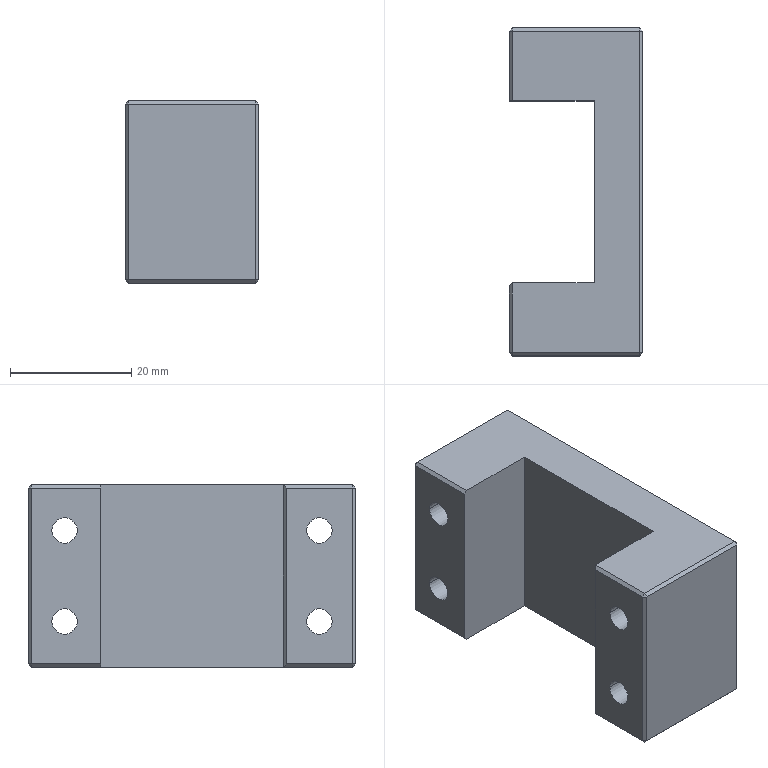Component | SolidWorks | XM-WST05-2009-3 | 1 solid | 41 faces | box 22 x 54 x 30 mm | volume 21772 mm3 | plane 33 | cylinder 8 | commonest cylinder face diameters 4.2 x8
build123d program:
from build123d import *

# Parameters (mm, degrees)
SKETCH1_W           = 54
SKETCH1_H           = 30
BOSS_EXTRUDE1_DEPTH = 22
SKETCH2_W           = 30
SKETCH2_H           = 28
CUT_EXTRUDE1_DEPTH  = 46.967
M5_TAPPED_HOLE1_D   = 4.2
CHAMFER1_SIZE       = 0.5


with BuildPart() as part:
    # Sketch1 → Boss-Extrude1 (new body)
    with BuildSketch(Plane.XY):
        Rectangle(SKETCH1_W, SKETCH1_H)
    extrude(amount=BOSS_EXTRUDE1_DEPTH)

    # Sketch2 → Cut-Extrude1 (cut, through all)
    with BuildSketch(Plane(origin=(0, 15, 0), x_dir=(1, 0, 0), z_dir=(0, 1, 0))):
        with Locations((0, -22)):
            Rectangle(SKETCH2_W, SKETCH2_H)
    extrude(amount=-CUT_EXTRUDE1_DEPTH, mode=Mode.SUBTRACT)

    # M5 Tapped Hole1 (through all)
    with Locations(Plane.XY.offset(22)):
        with Locations((-21, -7.5), (-21, 7.5), (21, 7.5), (21, -7.5)):
            Hole(M5_TAPPED_HOLE1_D / 2)

    # Chamfer1
    chamfer1_edges = [part.edges().sort_by_distance(p)[0] for p in [
        (27, 0, 22),
        (21, 15, 22),
        (21, -15, 22),
        (-21, 15, 22),
        (15, 0, 22),
        (-27, 0, 22),
        (0, 15, 0),
        (27, 0, 0),
        (0, -15, 0),
        (-27, 0, 0),
        (-21, -15, 22),
        (-27, 15, 11),
        (27, 15, 11),
        (27, -15, 11),
        (-27, -15, 11),
    ]]
    chamfer(chamfer1_edges, length=CHAMFER1_SIZE)


solid = part.part

# Placed as in the assembly
solid = solid.moved(Location((-131.071, 48.669, 455.899), (90, -90, 0)))
STEP:
#1=COLOUR_RGB('',0.7922,0.8196,0.9333);
#2=FILL_AREA_STYLE_COLOUR('',#1);
#3=FILL_AREA_STYLE('',(#2));
#4=SURFACE_STYLE_FILL_AREA(#3);
#5=SURFACE_SIDE_STYLE('',(#4));
#6=SURFACE_STYLE_USAGE(.BOTH.,#5);
#7=PRESENTATION_STYLE_ASSIGNMENT((#6));
#8=CARTESIAN_POINT('',(-5.16,2.826,17.654));
#9=VERTEX_POINT('',#8);
#10=CARTESIAN_POINT('',(-5.16,2.66,17.654));
#11=VERTEX_POINT('',#10);
#12=CARTESIAN_POINT('',(-5.16,2.743,17.654));
#13=DIRECTION('',(-1.,0.,-0.));
#14=DIRECTION('',(0.,-1.,0.));
#15=AXIS2_PLACEMENT_3D('',#12,#13,#14);
#16=CIRCLE('',#15,0.08268);
#17=EDGE_CURVE('',#9,#11,#16,.T.);
#18=ORIENTED_EDGE('',*,*,#17,.F.);
#19=CARTESIAN_POINT('',(-6.026,2.826,17.654));
#20=VERTEX_POINT('',#19);
#21=CARTESIAN_POINT('',(-6.026,2.826,17.654));
#22=DIRECTION('',(-1.,0.,-0.));
#23=VECTOR('',#22,39.37);
#24=LINE('',#21,#23);
#25=EDGE_CURVE('',#9,#20,#24,.T.);
#26=ORIENTED_EDGE('',*,*,#25,.T.);
#27=CARTESIAN_POINT('',(-6.026,2.66,17.654));
#28=VERTEX_POINT('',#27);
#29=CARTESIAN_POINT('',(-6.026,2.743,17.654));
#30=DIRECTION('',(-1.,0.,-0.));
#31=DIRECTION('',(0.,-1.,0.));
#32=AXIS2_PLACEMENT_3D('',#29,#30,#31);
#33=CIRCLE('',#32,0.08268);
#34=EDGE_CURVE('',#20,#28,#33,.T.);
#35=ORIENTED_EDGE('',*,*,#34,.T.);
#36=CARTESIAN_POINT('',(-6.026,2.66,17.654));
#37=DIRECTION('',(-1.,0.,-0.));
#38=VECTOR('',#37,39.37);
#39=LINE('',#36,#38);
#40=EDGE_CURVE('',#11,#28,#39,.T.);
#41=ORIENTED_EDGE('',*,*,#40,.F.);
#42=EDGE_LOOP('',(#18,#26,#35,#41));
#43=FACE_OUTER_BOUND('',#42,.T.);
#44=CARTESIAN_POINT('',(-6.026,2.743,17.654));
#45=DIRECTION('',(-1.,0.,-0.));
#46=DIRECTION('',(0.,-1.,0.));
#47=AXIS2_PLACEMENT_3D('',#44,#45,#46);
#48=CYLINDRICAL_SURFACE('',#47,0.08268);
#49=ADVANCED_FACE('',(#43),#48,.F.);
#50=CARTESIAN_POINT('',(-5.16,2.826,18.244));
#51=VERTEX_POINT('',#50);
#52=CARTESIAN_POINT('',(-5.16,2.66,18.244));
#53=VERTEX_POINT('',#52);
#54=CARTESIAN_POINT('',(-5.16,2.743,18.244));
#55=DIRECTION('',(-1.,0.,-0.));
#56=DIRECTION('',(0.,-1.,0.));
#57=AXIS2_PLACEMENT_3D('',#54,#55,#56);
#58=CIRCLE('',#57,0.08268);
#59=EDGE_CURVE('',#51,#53,#58,.T.);
#60=ORIENTED_EDGE('',*,*,#59,.F.);
#61=CARTESIAN_POINT('',(-6.026,2.826,18.244));
#62=VERTEX_POINT('',#61);
#63=CARTESIAN_POINT('',(-6.026,2.826,18.244));
#64=DIRECTION('',(-1.,0.,-0.));
#65=VECTOR('',#64,39.37);
#66=LINE('',#63,#65);
#67=EDGE_CURVE('',#51,#62,#66,.T.);
#68=ORIENTED_EDGE('',*,*,#67,.T.);
#69=CARTESIAN_POINT('',(-6.026,2.66,18.244));
#70=VERTEX_POINT('',#69);
#71=CARTESIAN_POINT('',(-6.026,2.743,18.244));
#72=DIRECTION('',(-1.,0.,-0.));
#73=DIRECTION('',(0.,-1.,0.));
#74=AXIS2_PLACEMENT_3D('',#71,#72,#73);
#75=CIRCLE('',#74,0.08268);
#76=EDGE_CURVE('',#62,#70,#75,.T.);
#77=ORIENTED_EDGE('',*,*,#76,.T.);
#78=CARTESIAN_POINT('',(-6.026,2.66,18.244));
#79=DIRECTION('',(-1.,0.,-0.));
#80=VECTOR('',#79,39.37);
#81=LINE('',#78,#80);
#82=EDGE_CURVE('',#53,#70,#81,.T.);
#83=ORIENTED_EDGE('',*,*,#82,.F.);
#84=EDGE_LOOP('',(#60,#68,#77,#83));
#85=FACE_OUTER_BOUND('',#84,.T.);
#86=CARTESIAN_POINT('',(-6.026,2.743,18.244));
#87=DIRECTION('',(-1.,0.,-0.));
#88=DIRECTION('',(0.,-1.,0.));
#89=AXIS2_PLACEMENT_3D('',#86,#87,#88);
#90=CYLINDRICAL_SURFACE('',#89,0.08268);
#91=ADVANCED_FACE('',(#85),#90,.F.);
#92=CARTESIAN_POINT('',(-5.16,1.172,18.244));
#93=VERTEX_POINT('',#92);
#94=CARTESIAN_POINT('',(-5.16,1.007,18.244));
#95=VERTEX_POINT('',#94);
#96=CARTESIAN_POINT('',(-5.16,1.089,18.244));
#97=DIRECTION('',(-1.,0.,-0.));
#98=DIRECTION('',(0.,-1.,0.));
#99=AXIS2_PLACEMENT_3D('',#96,#97,#98);
#100=CIRCLE('',#99,0.08268);
#101=EDGE_CURVE('',#93,#95,#100,.T.);
#102=ORIENTED_EDGE('',*,*,#101,.F.);
#103=CARTESIAN_POINT('',(-6.026,1.172,18.244));
#104=VERTEX_POINT('',#103);
#105=CARTESIAN_POINT('',(-6.026,1.172,18.244));
#106=DIRECTION('',(-1.,0.,-0.));
#107=VECTOR('',#106,39.37);
#108=LINE('',#105,#107);
#109=EDGE_CURVE('',#93,#104,#108,.T.);
#110=ORIENTED_EDGE('',*,*,#109,.T.);
#111=CARTESIAN_POINT('',(-6.026,1.007,18.244));
#112=VERTEX_POINT('',#111);
#113=CARTESIAN_POINT('',(-6.026,1.089,18.244));
#114=DIRECTION('',(-1.,0.,-0.));
#115=DIRECTION('',(0.,-1.,0.));
#116=AXIS2_PLACEMENT_3D('',#113,#114,#115);
#117=CIRCLE('',#116,0.08268);
#118=EDGE_CURVE('',#104,#112,#117,.T.);
#119=ORIENTED_EDGE('',*,*,#118,.T.);
#120=CARTESIAN_POINT('',(-6.026,1.007,18.244));
#121=DIRECTION('',(-1.,0.,-0.));
#122=VECTOR('',#121,39.37);
#123=LINE('',#120,#122);
#124=EDGE_CURVE('',#95,#112,#123,.T.);
#125=ORIENTED_EDGE('',*,*,#124,.F.);
#126=EDGE_LOOP('',(#102,#110,#119,#125));
#127=FACE_OUTER_BOUND('',#126,.T.);
#128=CARTESIAN_POINT('',(-6.026,1.089,18.244));
#129=DIRECTION('',(-1.,0.,-0.));
#130=DIRECTION('',(0.,-1.,0.));
#131=AXIS2_PLACEMENT_3D('',#128,#129,#130);
#132=CYLINDRICAL_SURFACE('',#131,0.08268);
#133=ADVANCED_FACE('',(#127),#132,.F.);
#134=CARTESIAN_POINT('',(-5.16,1.172,17.654));
#135=VERTEX_POINT('',#134);
#136=CARTESIAN_POINT('',(-5.16,1.007,17.654));
#137=VERTEX_POINT('',#136);
#138=CARTESIAN_POINT('',(-5.16,1.089,17.654));
#139=DIRECTION('',(-1.,0.,-0.));
#140=DIRECTION('',(0.,-1.,0.));
#141=AXIS2_PLACEMENT_3D('',#138,#139,#140);
#142=CIRCLE('',#141,0.08268);
#143=EDGE_CURVE('',#135,#137,#142,.T.);
#144=ORIENTED_EDGE('',*,*,#143,.F.);
#145=CARTESIAN_POINT('',(-6.026,1.172,17.654));
#146=VERTEX_POINT('',#145);
#147=CARTESIAN_POINT('',(-6.026,1.172,17.654));
#148=DIRECTION('',(-1.,0.,-0.));
#149=VECTOR('',#148,39.37);
#150=LINE('',#147,#149);
#151=EDGE_CURVE('',#135,#146,#150,.T.);
#152=ORIENTED_EDGE('',*,*,#151,.T.);
#153=CARTESIAN_POINT('',(-6.026,1.007,17.654));
#154=VERTEX_POINT('',#153);
#155=CARTESIAN_POINT('',(-6.026,1.089,17.654));
#156=DIRECTION('',(-1.,0.,-0.));
#157=DIRECTION('',(0.,-1.,0.));
#158=AXIS2_PLACEMENT_3D('',#155,#156,#157);
#159=CIRCLE('',#158,0.08268);
#160=EDGE_CURVE('',#146,#154,#159,.T.);
#161=ORIENTED_EDGE('',*,*,#160,.T.);
#162=CARTESIAN_POINT('',(-6.026,1.007,17.654));
#163=DIRECTION('',(-1.,0.,-0.));
#164=VECTOR('',#163,39.37);
#165=LINE('',#162,#164);
#166=EDGE_CURVE('',#137,#154,#165,.T.);
#167=ORIENTED_EDGE('',*,*,#166,.F.);
#168=EDGE_LOOP('',(#144,#152,#161,#167));
#169=FACE_OUTER_BOUND('',#168,.T.);
#170=CARTESIAN_POINT('',(-6.026,1.089,17.654));
#171=DIRECTION('',(-1.,0.,-0.));
#172=DIRECTION('',(0.,-1.,0.));
#173=AXIS2_PLACEMENT_3D('',#170,#171,#172);
#174=CYLINDRICAL_SURFACE('',#173,0.08268);
#175=ADVANCED_FACE('',(#169),#174,.F.);
#176=CARTESIAN_POINT('',(-6.026,2.743,17.654));
#177=DIRECTION('',(-1.,0.,-0.));
#178=DIRECTION('',(0.,-1.,0.));
#179=AXIS2_PLACEMENT_3D('',#176,#177,#178);
#180=CIRCLE('',#179,0.08268);
#181=EDGE_CURVE('',#28,#20,#180,.T.);
#182=ORIENTED_EDGE('',*,*,#181,.F.);
#183=ORIENTED_EDGE('',*,*,#34,.F.);
#184=EDGE_LOOP('',(#182,#183));
#185=FACE_BOUND('',#184,.T.);
#186=CARTESIAN_POINT('',(-6.026,2.743,18.244));
#187=DIRECTION('',(-1.,0.,-0.));
#188=DIRECTION('',(0.,-1.,0.));
#189=AXIS2_PLACEMENT_3D('',#186,#187,#188);
#190=CIRCLE('',#189,0.08268);
#191=EDGE_CURVE('',#70,#62,#190,.T.);
#192=ORIENTED_EDGE('',*,*,#191,.F.);
#193=ORIENTED_EDGE('',*,*,#76,.F.);
#194=EDGE_LOOP('',(#192,#193));
#195=FACE_BOUND('',#194,.T.);
#196=CARTESIAN_POINT('',(-6.026,2.507,17.378));
#197=VERTEX_POINT('',#196);
#198=CARTESIAN_POINT('',(-6.026,2.507,18.52));
#199=VERTEX_POINT('',#198);
#200=CARTESIAN_POINT('',(-6.026,2.507,17.358));
#201=DIRECTION('',(-0.,0.,1.));
#202=VECTOR('',#201,39.37);
#203=LINE('',#200,#202);
#204=EDGE_CURVE('',#197,#199,#203,.T.);
#205=ORIENTED_EDGE('',*,*,#204,.T.);
#206=CARTESIAN_POINT('',(-6.026,2.959,18.52));
#207=VERTEX_POINT('',#206);
#208=CARTESIAN_POINT('',(-6.026,2.979,18.52));
#209=DIRECTION('',(0.,1.,-0.));
#210=VECTOR('',#209,39.37);
#211=LINE('',#208,#210);
#212=EDGE_CURVE('',#199,#207,#211,.T.);
#213=ORIENTED_EDGE('',*,*,#212,.T.);
#214=CARTESIAN_POINT('',(-6.026,2.959,17.378));
#215=VERTEX_POINT('',#214);
#216=CARTESIAN_POINT('',(-6.026,2.959,17.358));
#217=DIRECTION('',(0.,-0.,-1.));
#218=VECTOR('',#217,39.37);
#219=LINE('',#216,#218);
#220=EDGE_CURVE('',#207,#215,#219,.T.);
#221=ORIENTED_EDGE('',*,*,#220,.T.);
#222=CARTESIAN_POINT('',(-6.026,2.979,17.378));
#223=DIRECTION('',(-0.,-1.,0.));
#224=VECTOR('',#223,39.37);
#225=LINE('',#222,#224);
#226=EDGE_CURVE('',#215,#197,#225,.T.);
#227=ORIENTED_EDGE('',*,*,#226,.T.);
#228=EDGE_LOOP('',(#205,#213,#221,#227));
#229=FACE_OUTER_BOUND('',#228,.T.);
#230=CARTESIAN_POINT('',(-6.026,2.979,17.358));
#231=DIRECTION('',(1.,-0.,0.));
#232=DIRECTION('',(0.,1.,-0.));
#233=AXIS2_PLACEMENT_3D('',#230,#231,#232);
#234=PLANE('',#233);
#235=ADVANCED_FACE('',(#185,#195,#229),#234,.F.);
#236=CARTESIAN_POINT('',(-6.007,2.979,17.378));
#237=VERTEX_POINT('',#236);
#238=CARTESIAN_POINT('',(-6.007,2.979,18.52));
#239=VERTEX_POINT('',#238);
#240=CARTESIAN_POINT('',(-6.007,2.979,18.539));
#241=DIRECTION('',(-0.,0.,1.));
#242=VECTOR('',#241,39.37);
#243=LINE('',#240,#242);
#244=EDGE_CURVE('',#237,#239,#243,.T.);
#245=ORIENTED_EDGE('',*,*,#244,.T.);
#246=CARTESIAN_POINT('',(-5.18,2.979,18.52));
#247=VERTEX_POINT('',#246);
#248=CARTESIAN_POINT('',(-6.026,2.979,18.52));
#249=DIRECTION('',(1.,-0.,0.));
#250=VECTOR('',#249,39.37);
#251=LINE('',#248,#250);
#252=EDGE_CURVE('',#239,#247,#251,.T.);
#253=ORIENTED_EDGE('',*,*,#252,.T.);
#254=CARTESIAN_POINT('',(-5.18,2.979,17.378));
#255=VERTEX_POINT('',#254);
#256=CARTESIAN_POINT('',(-5.18,2.979,17.358));
#257=DIRECTION('',(0.,-0.,-1.));
#258=VECTOR('',#257,39.37);
#259=LINE('',#256,#258);
#260=EDGE_CURVE('',#247,#255,#259,.T.);
#261=ORIENTED_EDGE('',*,*,#260,.T.);
#262=CARTESIAN_POINT('',(-6.026,2.979,17.378));
#263=DIRECTION('',(-1.,0.,-0.));
#264=VECTOR('',#263,39.37);
#265=LINE('',#262,#264);
#266=EDGE_CURVE('',#255,#237,#265,.T.);
#267=ORIENTED_EDGE('',*,*,#266,.T.);
#268=EDGE_LOOP('',(#245,#253,#261,#267));
#269=FACE_OUTER_BOUND('',#268,.T.);
#270=CARTESIAN_POINT('',(-6.026,2.979,18.539));
#271=DIRECTION('',(-0.,-1.,0.));
#272=DIRECTION('',(-0.,0.,1.));
#273=AXIS2_PLACEMENT_3D('',#270,#271,#272);
#274=PLANE('',#273);
#275=ADVANCED_FACE('',(#269),#274,.F.);
#276=CARTESIAN_POINT('',(-5.18,0.8728,17.358));
#277=VERTEX_POINT('',#276);
#278=CARTESIAN_POINT('',(-6.007,0.8728,17.358));
#279=VERTEX_POINT('',#278);
#280=CARTESIAN_POINT('',(-6.026,0.8728,17.358));
#281=DIRECTION('',(-1.,0.,-0.));
#282=VECTOR('',#281,39.37);
#283=LINE('',#280,#282);
#284=EDGE_CURVE('',#277,#279,#283,.T.);
#285=ORIENTED_EDGE('',*,*,#284,.T.);
#286=CARTESIAN_POINT('',(-6.007,1.326,17.358));
#287=VERTEX_POINT('',#286);
#288=CARTESIAN_POINT('',(-6.007,0.8531,17.358));
#289=DIRECTION('',(0.,1.,-0.));
#290=VECTOR('',#289,39.37);
#291=LINE('',#288,#290);
#292=EDGE_CURVE('',#279,#287,#291,.T.);
#293=ORIENTED_EDGE('',*,*,#292,.T.);
#294=CARTESIAN_POINT('',(-5.475,1.326,17.358));
#295=VERTEX_POINT('',#294);
#296=CARTESIAN_POINT('',(-6.578,1.326,17.358));
#297=DIRECTION('',(1.,-0.,0.));
#298=VECTOR('',#297,39.37);
#299=LINE('',#296,#298);
#300=EDGE_CURVE('',#287,#295,#299,.T.);
#301=ORIENTED_EDGE('',*,*,#300,.T.);
#302=CARTESIAN_POINT('',(-5.475,2.507,17.358));
#303=VERTEX_POINT('',#302);
#304=CARTESIAN_POINT('',(-5.475,1.326,17.358));
#305=DIRECTION('',(0.,1.,-0.));
#306=VECTOR('',#305,39.37);
#307=LINE('',#304,#306);
#308=EDGE_CURVE('',#295,#303,#307,.T.);
#309=ORIENTED_EDGE('',*,*,#308,.T.);
#310=CARTESIAN_POINT('',(-6.007,2.507,17.358));
#311=VERTEX_POINT('',#310);
#312=CARTESIAN_POINT('',(-6.578,2.507,17.358));
#313=DIRECTION('',(-1.,0.,-0.));
#314=VECTOR('',#313,39.37);
#315=LINE('',#312,#314);
#316=EDGE_CURVE('',#303,#311,#315,.T.);
#317=ORIENTED_EDGE('',*,*,#316,.T.);
#318=CARTESIAN_POINT('',(-6.007,2.959,17.358));
#319=VERTEX_POINT('',#318);
#320=CARTESIAN_POINT('',(-6.007,0.8531,17.358));
#321=DIRECTION('',(0.,1.,-0.));
#322=VECTOR('',#321,39.37);
#323=LINE('',#320,#322);
#324=EDGE_CURVE('',#311,#319,#323,.T.);
#325=ORIENTED_EDGE('',*,*,#324,.T.);
#326=CARTESIAN_POINT('',(-5.18,2.959,17.358));
#327=VERTEX_POINT('',#326);
#328=CARTESIAN_POINT('',(-6.026,2.959,17.358));
#329=DIRECTION('',(1.,-0.,0.));
#330=VECTOR('',#329,39.37);
#331=LINE('',#328,#330);
#332=EDGE_CURVE('',#319,#327,#331,.T.);
#333=ORIENTED_EDGE('',*,*,#332,.T.);
#334=CARTESIAN_POINT('',(-5.18,0.8531,17.358));
#335=DIRECTION('',(-0.,-1.,0.));
#336=VECTOR('',#335,39.37);
#337=LINE('',#334,#336);
#338=EDGE_CURVE('',#327,#277,#337,.T.);
#339=ORIENTED_EDGE('',*,*,#338,.T.);
#340=EDGE_LOOP('',(#285,#293,#301,#309,#317,#325,#333,#339));
#341=FACE_OUTER_BOUND('',#340,.T.);
#342=CARTESIAN_POINT('',(-6.026,0.8531,17.358));
#343=DIRECTION('',(-0.,0.,1.));
#344=DIRECTION('',(0.,1.,-0.));
#345=AXIS2_PLACEMENT_3D('',#342,#343,#344);
#346=PLANE('',#345);
#347=ADVANCED_FACE('',(#341),#346,.F.);
#348=CARTESIAN_POINT('',(-6.007,0.8531,18.52));
#349=VERTEX_POINT('',#348);
#350=CARTESIAN_POINT('',(-6.007,0.8531,17.378));
#351=VERTEX_POINT('',#350);
#352=CARTESIAN_POINT('',(-6.007,0.8531,18.539));
#353=DIRECTION('',(0.,-0.,-1.));
#354=VECTOR('',#353,39.37);
#355=LINE('',#352,#354);
#356=EDGE_CURVE('',#349,#351,#355,.T.);
#357=ORIENTED_EDGE('',*,*,#356,.T.);
#358=CARTESIAN_POINT('',(-5.18,0.8531,17.378));
#359=VERTEX_POINT('',#358);
#360=CARTESIAN_POINT('',(-6.026,0.8531,17.378));
#361=DIRECTION('',(1.,-0.,0.));
#362=VECTOR('',#361,39.37);
#363=LINE('',#360,#362);
#364=EDGE_CURVE('',#351,#359,#363,.T.);
#365=ORIENTED_EDGE('',*,*,#364,.T.);
#366=CARTESIAN_POINT('',(-5.18,0.8531,18.52));
#367=VERTEX_POINT('',#366);
#368=CARTESIAN_POINT('',(-5.18,0.8531,18.539));
#369=DIRECTION('',(-0.,0.,1.));
#370=VECTOR('',#369,39.37);
#371=LINE('',#368,#370);
#372=EDGE_CURVE('',#359,#367,#371,.T.);
#373=ORIENTED_EDGE('',*,*,#372,.T.);
#374=CARTESIAN_POINT('',(-6.026,0.8531,18.52));
#375=DIRECTION('',(-1.,0.,-0.));
#376=VECTOR('',#375,39.37);
#377=LINE('',#374,#376);
#378=EDGE_CURVE('',#367,#349,#377,.T.);
#379=ORIENTED_EDGE('',*,*,#378,.T.);
#380=EDGE_LOOP('',(#357,#365,#373,#379));
#381=FACE_OUTER_BOUND('',#380,.T.);
#382=CARTESIAN_POINT('',(-6.026,0.8531,18.539));
#383=DIRECTION('',(0.,1.,-0.));
#384=DIRECTION('',(0.,-0.,-1.));
#385=AXIS2_PLACEMENT_3D('',#382,#383,#384);
#386=PLANE('',#385);
#387=ADVANCED_FACE('',(#381),#386,.F.);
#388=CARTESIAN_POINT('',(-5.18,2.959,18.539));
#389=VERTEX_POINT('',#388);
#390=CARTESIAN_POINT('',(-6.007,2.959,18.539));
#391=VERTEX_POINT('',#390);
#392=CARTESIAN_POINT('',(-6.026,2.959,18.539));
#393=DIRECTION('',(-1.,0.,-0.));
#394=VECTOR('',#393,39.37);
#395=LINE('',#392,#394);
#396=EDGE_CURVE('',#389,#391,#395,.T.);
#397=ORIENTED_EDGE('',*,*,#396,.T.);
#398=CARTESIAN_POINT('',(-6.007,2.507,18.539));
#399=VERTEX_POINT('',#398);
#400=CARTESIAN_POINT('',(-6.007,0.8531,18.539));
#401=DIRECTION('',(-0.,-1.,0.));
#402=VECTOR('',#401,39.37);
#403=LINE('',#400,#402);
#404=EDGE_CURVE('',#391,#399,#403,.T.);
#405=ORIENTED_EDGE('',*,*,#404,.T.);
#406=CARTESIAN_POINT('',(-5.475,2.507,18.539));
#407=VERTEX_POINT('',#406);
#408=CARTESIAN_POINT('',(-6.578,2.507,18.539));
#409=DIRECTION('',(-1.,0.,-0.));
#410=VECTOR('',#409,39.37);
#411=LINE('',#408,#410);
#412=EDGE_CURVE('',#407,#399,#411,.T.);
#413=ORIENTED_EDGE('',*,*,#412,.F.);
#414=CARTESIAN_POINT('',(-5.475,1.326,18.539));
#415=VERTEX_POINT('',#414);
#416=CARTESIAN_POINT('',(-5.475,1.326,18.539));
#417=DIRECTION('',(0.,1.,-0.));
#418=VECTOR('',#417,39.37);
#419=LINE('',#416,#418);
#420=EDGE_CURVE('',#415,#407,#419,.T.);
#421=ORIENTED_EDGE('',*,*,#420,.F.);
#422=CARTESIAN_POINT('',(-6.007,1.326,18.539));
#423=VERTEX_POINT('',#422);
#424=CARTESIAN_POINT('',(-6.578,1.326,18.539));
#425=DIRECTION('',(1.,-0.,0.));
#426=VECTOR('',#425,39.37);
#427=LINE('',#424,#426);
#428=EDGE_CURVE('',#423,#415,#427,.T.);
#429=ORIENTED_EDGE('',*,*,#428,.F.);
#430=CARTESIAN_POINT('',(-6.007,0.8728,18.539));
#431=VERTEX_POINT('',#430);
#432=CARTESIAN_POINT('',(-6.007,0.8531,18.539));
#433=DIRECTION('',(-0.,-1.,0.));
#434=VECTOR('',#433,39.37);
#435=LINE('',#432,#434);
#436=EDGE_CURVE('',#423,#431,#435,.T.);
#437=ORIENTED_EDGE('',*,*,#436,.T.);
#438=CARTESIAN_POINT('',(-5.18,0.8728,18.539));
#439=VERTEX_POINT('',#438);
#440=CARTESIAN_POINT('',(-6.026,0.8728,18.539));
#441=DIRECTION('',(1.,-0.,0.));
#442=VECTOR('',#441,39.37);
#443=LINE('',#440,#442);
#444=EDGE_CURVE('',#431,#439,#443,.T.);
#445=ORIENTED_EDGE('',*,*,#444,.T.);
#446=CARTESIAN_POINT('',(-5.18,2.979,18.539));
#447=DIRECTION('',(0.,1.,-0.));
#448=VECTOR('',#447,39.37);
#449=LINE('',#446,#448);
#450=EDGE_CURVE('',#439,#389,#449,.T.);
#451=ORIENTED_EDGE('',*,*,#450,.T.);
#452=EDGE_LOOP('',(#397,#405,#413,#421,#429,#437,#445,#451));
#453=FACE_OUTER_BOUND('',#452,.T.);
#454=CARTESIAN_POINT('',(-6.026,0.8531,18.539));
#455=DIRECTION('',(0.,-0.,-1.));
#456=DIRECTION('',(-0.,-1.,0.));
#457=AXIS2_PLACEMENT_3D('',#454,#455,#456);
#458=PLANE('',#457);
#459=ADVANCED_FACE('',(#453),#458,.F.);
#460=CARTESIAN_POINT('',(-6.026,1.306,17.378));
#461=VERTEX_POINT('',#460);
#462=CARTESIAN_POINT('',(-6.026,0.8728,17.378));
#463=VERTEX_POINT('',#462);
#464=CARTESIAN_POINT('',(-6.026,2.979,17.378));
#465=DIRECTION('',(-0.,-1.,0.));
#466=VECTOR('',#465,39.37);
#467=LINE('',#464,#466);
#468=EDGE_CURVE('',#461,#463,#467,.T.);
#469=ORIENTED_EDGE('',*,*,#468,.T.);
#470=CARTESIAN_POINT('',(-6.026,0.8728,18.52));
#471=VERTEX_POINT('',#470);
#472=CARTESIAN_POINT('',(-6.026,0.8728,17.358));
#473=DIRECTION('',(-0.,0.,1.));
#474=VECTOR('',#473,39.37);
#475=LINE('',#472,#474);
#476=EDGE_CURVE('',#463,#471,#475,.T.);
#477=ORIENTED_EDGE('',*,*,#476,.T.);
#478=CARTESIAN_POINT('',(-6.026,1.306,18.52));
#479=VERTEX_POINT('',#478);
#480=CARTESIAN_POINT('',(-6.026,2.979,18.52));
#481=DIRECTION('',(0.,1.,-0.));
#482=VECTOR('',#481,39.37);
#483=LINE('',#480,#482);
#484=EDGE_CURVE('',#471,#479,#483,.T.);
#485=ORIENTED_EDGE('',*,*,#484,.T.);
#486=CARTESIAN_POINT('',(-6.026,1.306,17.358));
#487=DIRECTION('',(0.,-0.,-1.));
#488=VECTOR('',#487,39.37);
#489=LINE('',#486,#488);
#490=EDGE_CURVE('',#479,#461,#489,.T.);
#491=ORIENTED_EDGE('',*,*,#490,.T.);
#492=EDGE_LOOP('',(#469,#477,#485,#491));
#493=FACE_OUTER_BOUND('',#492,.T.);
#494=CARTESIAN_POINT('',(-6.026,1.089,18.244));
#495=DIRECTION('',(-1.,0.,-0.));
#496=DIRECTION('',(0.,-1.,0.));
#497=AXIS2_PLACEMENT_3D('',#494,#495,#496);
#498=CIRCLE('',#497,0.08268);
#499=EDGE_CURVE('',#112,#104,#498,.T.);
#500=ORIENTED_EDGE('',*,*,#499,.F.);
#501=ORIENTED_EDGE('',*,*,#118,.F.);
#502=EDGE_LOOP('',(#500,#501));
#503=FACE_BOUND('',#502,.T.);
#504=CARTESIAN_POINT('',(-6.026,1.089,17.654));
#505=DIRECTION('',(-1.,0.,-0.));
#506=DIRECTION('',(0.,-1.,0.));
#507=AXIS2_PLACEMENT_3D('',#504,#505,#506);
#508=CIRCLE('',#507,0.08268);
#509=EDGE_CURVE('',#154,#146,#508,.T.);
#510=ORIENTED_EDGE('',*,*,#509,.F.);
#511=ORIENTED_EDGE('',*,*,#160,.F.);
#512=EDGE_LOOP('',(#510,#511));
#513=FACE_BOUND('',#512,.T.);
#514=CARTESIAN_POINT('',(-6.026,2.979,17.358));
#515=DIRECTION('',(1.,-0.,0.));
#516=DIRECTION('',(0.,1.,-0.));
#517=AXIS2_PLACEMENT_3D('',#514,#515,#516);
#518=PLANE('',#517);
#519=ADVANCED_FACE('',(#493,#503,#513),#518,.F.);
#520=CARTESIAN_POINT('',(-5.16,2.959,18.52));
#521=VERTEX_POINT('',#520);
#522=CARTESIAN_POINT('',(-5.16,0.8728,18.52));
#523=VERTEX_POINT('',#522);
#524=CARTESIAN_POINT('',(-5.16,0.8531,18.52));
#525=DIRECTION('',(-0.,-1.,0.));
#526=VECTOR('',#525,39.37);
#527=LINE('',#524,#526);
#528=EDGE_CURVE('',#521,#523,#527,.T.);
#529=ORIENTED_EDGE('',*,*,#528,.T.);
#530=CARTESIAN_POINT('',(-5.16,0.8728,17.378));
#531=VERTEX_POINT('',#530);
#532=CARTESIAN_POINT('',(-5.16,0.8728,17.358));
#533=DIRECTION('',(0.,-0.,-1.));
#534=VECTOR('',#533,39.37);
#535=LINE('',#532,#534);
#536=EDGE_CURVE('',#523,#531,#535,.T.);
#537=ORIENTED_EDGE('',*,*,#536,.T.);
#538=CARTESIAN_POINT('',(-5.16,2.959,17.378));
#539=VERTEX_POINT('',#538);
#540=CARTESIAN_POINT('',(-5.16,2.979,17.378));
#541=DIRECTION('',(0.,1.,-0.));
#542=VECTOR('',#541,39.37);
#543=LINE('',#540,#542);
#544=EDGE_CURVE('',#531,#539,#543,.T.);
#545=ORIENTED_EDGE('',*,*,#544,.T.);
#546=CARTESIAN_POINT('',(-5.16,2.959,18.539));
#547=DIRECTION('',(-0.,0.,1.));
#548=VECTOR('',#547,39.37);
#549=LINE('',#546,#548);
#550=EDGE_CURVE('',#539,#521,#549,.T.);
#551=ORIENTED_EDGE('',*,*,#550,.T.);
#552=EDGE_LOOP('',(#529,#537,#545,#551));
#553=FACE_OUTER_BOUND('',#552,.T.);
#554=CARTESIAN_POINT('',(-5.16,2.743,17.654));
#555=DIRECTION('',(-1.,0.,-0.));
#556=DIRECTION('',(0.,-1.,0.));
#557=AXIS2_PLACEMENT_3D('',#554,#555,#556);
#558=CIRCLE('',#557,0.08268);
#559=EDGE_CURVE('',#11,#9,#558,.T.);
#560=ORIENTED_EDGE('',*,*,#559,.T.);
#561=ORIENTED_EDGE('',*,*,#17,.T.);
#562=EDGE_LOOP('',(#560,#561));
#563=FACE_BOUND('',#562,.T.);
#564=CARTESIAN_POINT('',(-5.16,2.743,18.244));
#565=DIRECTION('',(-1.,0.,-0.));
#566=DIRECTION('',(0.,-1.,0.));
#567=AXIS2_PLACEMENT_3D('',#564,#565,#566);
#568=CIRCLE('',#567,0.08268);
#569=EDGE_CURVE('',#53,#51,#568,.T.);
#570=ORIENTED_EDGE('',*,*,#569,.T.);
#571=ORIENTED_EDGE('',*,*,#59,.T.);
#572=EDGE_LOOP('',(#570,#571));
#573=FACE_BOUND('',#572,.T.);
#574=CARTESIAN_POINT('',(-5.16,1.089,18.244));
#575=DIRECTION('',(-1.,0.,-0.));
#576=DIRECTION('',(0.,-1.,0.));
#577=AXIS2_PLACEMENT_3D('',#574,#575,#576);
#578=CIRCLE('',#577,0.08268);
#579=EDGE_CURVE('',#95,#93,#578,.T.);
#580=ORIENTED_EDGE('',*,*,#579,.T.);
#581=ORIENTED_EDGE('',*,*,#101,.T.);
#582=EDGE_LOOP('',(#580,#581));
#583=FACE_BOUND('',#582,.T.);
#584=CARTESIAN_POINT('',(-5.16,1.089,17.654));
#585=DIRECTION('',(-1.,0.,-0.));
#586=DIRECTION('',(0.,-1.,0.));
#587=AXIS2_PLACEMENT_3D('',#584,#585,#586);
#588=CIRCLE('',#587,0.08268);
#589=EDGE_CURVE('',#137,#135,#588,.T.);
#590=ORIENTED_EDGE('',*,*,#589,.T.);
#591=ORIENTED_EDGE('',*,*,#143,.T.);
#592=EDGE_LOOP('',(#590,#591));
#593=FACE_BOUND('',#592,.T.);
#594=CARTESIAN_POINT('',(-5.16,2.979,17.358));
#595=DIRECTION('',(1.,-0.,0.));
#596=DIRECTION('',(0.,1.,-0.));
#597=AXIS2_PLACEMENT_3D('',#594,#595,#596);
#598=PLANE('',#597);
#599=ADVANCED_FACE('',(#553,#563,#573,#583,#593),#598,.T.);
#600=ORIENTED_EDGE('',*,*,#412,.T.);
#601=CARTESIAN_POINT('',(-6.026,2.507,18.52));
#602=DIRECTION('',(-0.7071,-0.,-0.7071));
#603=VECTOR('',#602,39.37);
#604=LINE('',#601,#603);
#605=EDGE_CURVE('',#399,#199,#604,.T.);
#606=ORIENTED_EDGE('',*,*,#605,.T.);
#607=ORIENTED_EDGE('',*,*,#204,.F.);
#608=CARTESIAN_POINT('',(-6.026,2.507,17.378));
#609=DIRECTION('',(0.7071,-0.,-0.7071));
#610=VECTOR('',#609,39.37);
#611=LINE('',#608,#610);
#612=EDGE_CURVE('',#197,#311,#611,.T.);
#613=ORIENTED_EDGE('',*,*,#612,.T.);
#614=ORIENTED_EDGE('',*,*,#316,.F.);
#615=CARTESIAN_POINT('',(-5.475,2.507,17.358));
#616=DIRECTION('',(-0.,0.,1.));
#617=VECTOR('',#616,39.37);
#618=LINE('',#615,#617);
#619=EDGE_CURVE('',#303,#407,#618,.T.);
#620=ORIENTED_EDGE('',*,*,#619,.T.);
#621=EDGE_LOOP('',(#600,#606,#607,#613,#614,#620));
#622=FACE_OUTER_BOUND('',#621,.T.);
#623=CARTESIAN_POINT('',(-6.578,2.507,17.358));
#624=DIRECTION('',(0.,1.,-0.));
#625=DIRECTION('',(0.,-0.,-1.));
#626=AXIS2_PLACEMENT_3D('',#623,#624,#625);
#627=PLANE('',#626);
#628=ADVANCED_FACE('',(#622),#627,.F.);
#629=ORIENTED_EDGE('',*,*,#300,.F.);
#630=CARTESIAN_POINT('',(-6.007,1.326,17.358));
#631=DIRECTION('',(-0.,0.,1.));
#632=VECTOR('',#631,39.37);
#633=LINE('',#630,#632);
#634=EDGE_CURVE('',#287,#423,#633,.T.);
#635=ORIENTED_EDGE('',*,*,#634,.T.);
#636=ORIENTED_EDGE('',*,*,#428,.T.);
#637=CARTESIAN_POINT('',(-5.475,1.326,17.358));
#638=DIRECTION('',(-0.,0.,1.));
#639=VECTOR('',#638,39.37);
#640=LINE('',#637,#639);
#641=EDGE_CURVE('',#295,#415,#640,.T.);
#642=ORIENTED_EDGE('',*,*,#641,.F.);
#643=EDGE_LOOP('',(#629,#635,#636,#642));
#644=FACE_OUTER_BOUND('',#643,.T.);
#645=CARTESIAN_POINT('',(-6.578,1.326,17.358));
#646=DIRECTION('',(-0.,-1.,0.));
#647=DIRECTION('',(-0.,0.,1.));
#648=AXIS2_PLACEMENT_3D('',#645,#646,#647);
#649=PLANE('',#648);
#650=ADVANCED_FACE('',(#644),#649,.F.);
#651=ORIENTED_EDGE('',*,*,#420,.T.);
#652=ORIENTED_EDGE('',*,*,#619,.F.);
#653=ORIENTED_EDGE('',*,*,#308,.F.);
#654=ORIENTED_EDGE('',*,*,#641,.T.);
#655=EDGE_LOOP('',(#651,#652,#653,#654));
#656=FACE_OUTER_BOUND('',#655,.T.);
#657=CARTESIAN_POINT('',(-5.475,1.326,17.358));
#658=DIRECTION('',(1.,-0.,0.));
#659=DIRECTION('',(0.,1.,-0.));
#660=AXIS2_PLACEMENT_3D('',#657,#658,#659);
#661=PLANE('',#660);
#662=ADVANCED_FACE('',(#656),#661,.F.);
#663=ORIENTED_EDGE('',*,*,#151,.F.);
#664=ORIENTED_EDGE('',*,*,#589,.F.);
#665=ORIENTED_EDGE('',*,*,#166,.T.);
#666=ORIENTED_EDGE('',*,*,#509,.T.);
#667=EDGE_LOOP('',(#663,#664,#665,#666));
#668=FACE_OUTER_BOUND('',#667,.T.);
#669=CARTESIAN_POINT('',(-6.026,1.089,17.654));
#670=DIRECTION('',(-1.,0.,-0.));
#671=DIRECTION('',(0.,-1.,0.));
#672=AXIS2_PLACEMENT_3D('',#669,#670,#671);
#673=CYLINDRICAL_SURFACE('',#672,0.08268);
#674=ADVANCED_FACE('',(#668),#673,.F.);
#675=ORIENTED_EDGE('',*,*,#109,.F.);
#676=ORIENTED_EDGE('',*,*,#579,.F.);
#677=ORIENTED_EDGE('',*,*,#124,.T.);
#678=ORIENTED_EDGE('',*,*,#499,.T.);
#679=EDGE_LOOP('',(#675,#676,#677,#678));
#680=FACE_OUTER_BOUND('',#679,.T.);
#681=CARTESIAN_POINT('',(-6.026,1.089,18.244));
#682=DIRECTION('',(-1.,0.,-0.));
#683=DIRECTION('',(0.,-1.,0.));
#684=AXIS2_PLACEMENT_3D('',#681,#682,#683);
#685=CYLINDRICAL_SURFACE('',#684,0.08268);
#686=ADVANCED_FACE('',(#680),#685,.F.);
#687=ORIENTED_EDGE('',*,*,#67,.F.);
#688=ORIENTED_EDGE('',*,*,#569,.F.);
#689=ORIENTED_EDGE('',*,*,#82,.T.);
#690=ORIENTED_EDGE('',*,*,#191,.T.);
#691=EDGE_LOOP('',(#687,#688,#689,#690));
#692=FACE_OUTER_BOUND('',#691,.T.);
#693=CARTESIAN_POINT('',(-6.026,2.743,18.244));
#694=DIRECTION('',(-1.,0.,-0.));
#695=DIRECTION('',(0.,-1.,0.));
#696=AXIS2_PLACEMENT_3D('',#693,#694,#695);
#697=CYLINDRICAL_SURFACE('',#696,0.08268);
#698=ADVANCED_FACE('',(#692),#697,.F.);
#699=ORIENTED_EDGE('',*,*,#25,.F.);
#700=ORIENTED_EDGE('',*,*,#559,.F.);
#701=ORIENTED_EDGE('',*,*,#40,.T.);
#702=ORIENTED_EDGE('',*,*,#181,.T.);
#703=EDGE_LOOP('',(#699,#700,#701,#702));
#704=FACE_OUTER_BOUND('',#703,.T.);
#705=CARTESIAN_POINT('',(-6.026,2.743,17.654));
#706=DIRECTION('',(-1.,0.,-0.));
#707=DIRECTION('',(0.,-1.,0.));
#708=AXIS2_PLACEMENT_3D('',#705,#706,#707);
#709=CYLINDRICAL_SURFACE('',#708,0.08268);
#710=ADVANCED_FACE('',(#704),#709,.F.);
#711=CARTESIAN_POINT('',(-6.007,2.959,18.539));
#712=DIRECTION('',(0.7071,-0.,0.7071));
#713=VECTOR('',#712,39.37);
#714=LINE('',#711,#713);
#715=EDGE_CURVE('',#207,#391,#714,.T.);
#716=ORIENTED_EDGE('',*,*,#715,.F.);
#717=ORIENTED_EDGE('',*,*,#212,.F.);
#718=ORIENTED_EDGE('',*,*,#605,.F.);
#719=ORIENTED_EDGE('',*,*,#404,.F.);
#720=EDGE_LOOP('',(#716,#717,#718,#719));
#721=FACE_OUTER_BOUND('',#720,.T.);
#722=CARTESIAN_POINT('',(-6.026,2.979,18.52));
#723=DIRECTION('',(0.7071,-0.,-0.7071));
#724=DIRECTION('',(0.7071,-0.,0.7071));
#725=AXIS2_PLACEMENT_3D('',#722,#723,#724);
#726=PLANE('',#725);
#727=ADVANCED_FACE('',(#721),#726,.F.);
#728=CARTESIAN_POINT('',(-6.017,2.969,18.52));
#729=DIRECTION('',(0.7071,0.7071,-0.));
#730=VECTOR('',#729,39.37);
#731=LINE('',#728,#730);
#732=EDGE_CURVE('',#207,#239,#731,.T.);
#733=ORIENTED_EDGE('',*,*,#732,.F.);
#734=ORIENTED_EDGE('',*,*,#715,.T.);
#735=CARTESIAN_POINT('',(-6.007,2.959,18.539));
#736=DIRECTION('',(-0.,-0.7071,0.7071));
#737=VECTOR('',#736,39.37);
#738=LINE('',#735,#737);
#739=EDGE_CURVE('',#239,#391,#738,.T.);
#740=ORIENTED_EDGE('',*,*,#739,.F.);
#741=EDGE_LOOP('',(#733,#734,#740));
#742=FACE_OUTER_BOUND('',#741,.T.);
#743=CARTESIAN_POINT('',(-6.007,2.959,18.539));
#744=DIRECTION('',(-0.5774,0.5774,0.5774));
#745=DIRECTION('',(0.,0.7071,-0.7071));
#746=AXIS2_PLACEMENT_3D('',#743,#744,#745);
#747=PLANE('',#746);
#748=ADVANCED_FACE('',(#742),#747,.T.);
#749=ORIENTED_EDGE('',*,*,#739,.T.);
#750=ORIENTED_EDGE('',*,*,#396,.F.);
#751=CARTESIAN_POINT('',(-5.18,2.979,18.52));
#752=DIRECTION('',(-0.,-0.7071,0.7071));
#753=VECTOR('',#752,39.37);
#754=LINE('',#751,#753);
#755=EDGE_CURVE('',#247,#389,#754,.T.);
#756=ORIENTED_EDGE('',*,*,#755,.F.);
#757=ORIENTED_EDGE('',*,*,#252,.F.);
#758=EDGE_LOOP('',(#749,#750,#756,#757));
#759=FACE_OUTER_BOUND('',#758,.T.);
#760=CARTESIAN_POINT('',(-6.026,2.979,18.52));
#761=DIRECTION('',(-0.,-0.7071,-0.7071));
#762=DIRECTION('',(-0.,-0.7071,0.7071));
#763=AXIS2_PLACEMENT_3D('',#760,#761,#762);
#764=PLANE('',#763);
#765=ADVANCED_FACE('',(#759),#764,.F.);
#766=ORIENTED_EDGE('',*,*,#732,.T.);
#767=ORIENTED_EDGE('',*,*,#244,.F.);
#768=CARTESIAN_POINT('',(-6.026,2.959,17.378));
#769=DIRECTION('',(0.7071,0.7071,-0.));
#770=VECTOR('',#769,39.37);
#771=LINE('',#768,#770);
#772=EDGE_CURVE('',#215,#237,#771,.T.);
#773=ORIENTED_EDGE('',*,*,#772,.F.);
#774=ORIENTED_EDGE('',*,*,#220,.F.);
#775=EDGE_LOOP('',(#766,#767,#773,#774));
#776=FACE_OUTER_BOUND('',#775,.T.);
#777=CARTESIAN_POINT('',(-6.026,2.959,17.358));
#778=DIRECTION('',(0.7071,-0.7071,0.));
#779=DIRECTION('',(0.7071,0.7071,-0.));
#780=AXIS2_PLACEMENT_3D('',#777,#778,#779);
#781=PLANE('',#780);
#782=ADVANCED_FACE('',(#776),#781,.F.);
#783=ORIENTED_EDGE('',*,*,#612,.F.);
#784=ORIENTED_EDGE('',*,*,#226,.F.);
#785=CARTESIAN_POINT('',(-6.026,2.959,17.378));
#786=DIRECTION('',(-0.7071,0.,0.7071));
#787=VECTOR('',#786,39.37);
#788=LINE('',#785,#787);
#789=EDGE_CURVE('',#319,#215,#788,.T.);
#790=ORIENTED_EDGE('',*,*,#789,.F.);
#791=ORIENTED_EDGE('',*,*,#324,.F.);
#792=EDGE_LOOP('',(#783,#784,#790,#791));
#793=FACE_OUTER_BOUND('',#792,.T.);
#794=CARTESIAN_POINT('',(-6.026,2.979,17.378));
#795=DIRECTION('',(0.7071,0.,0.7071));
#796=DIRECTION('',(-0.7071,0.,0.7071));
#797=AXIS2_PLACEMENT_3D('',#794,#795,#796);
#798=PLANE('',#797);
#799=ADVANCED_FACE('',(#793),#798,.F.);
#800=CARTESIAN_POINT('',(-5.18,2.979,18.52));
#801=DIRECTION('',(0.7071,-0.7071,0.));
#802=VECTOR('',#801,39.37);
#803=LINE('',#800,#802);
#804=EDGE_CURVE('',#247,#521,#803,.T.);
#805=ORIENTED_EDGE('',*,*,#804,.F.);
#806=ORIENTED_EDGE('',*,*,#755,.T.);
#807=CARTESIAN_POINT('',(-5.17,2.959,18.53));
#808=DIRECTION('',(-0.7071,-0.,0.7071));
#809=VECTOR('',#808,39.37);
#810=LINE('',#807,#809);
#811=EDGE_CURVE('',#521,#389,#810,.T.);
#812=ORIENTED_EDGE('',*,*,#811,.F.);
#813=EDGE_LOOP('',(#805,#806,#812));
#814=FACE_OUTER_BOUND('',#813,.T.);
#815=CARTESIAN_POINT('',(-5.18,2.979,18.52));
#816=DIRECTION('',(0.5774,0.5774,0.5774));
#817=DIRECTION('',(0.,0.7071,-0.7071));
#818=AXIS2_PLACEMENT_3D('',#815,#816,#817);
#819=PLANE('',#818);
#820=ADVANCED_FACE('',(#814),#819,.T.);
#821=ORIENTED_EDGE('',*,*,#789,.T.);
#822=ORIENTED_EDGE('',*,*,#772,.T.);
#823=CARTESIAN_POINT('',(-6.007,2.969,17.368));
#824=DIRECTION('',(0.,0.7071,0.7071));
#825=VECTOR('',#824,39.37);
#826=LINE('',#823,#825);
#827=EDGE_CURVE('',#319,#237,#826,.T.);
#828=ORIENTED_EDGE('',*,*,#827,.F.);
#829=EDGE_LOOP('',(#821,#822,#828));
#830=FACE_OUTER_BOUND('',#829,.T.);
#831=CARTESIAN_POINT('',(-6.026,2.959,17.378));
#832=DIRECTION('',(-0.5774,0.5774,-0.5774));
#833=DIRECTION('',(-0.7071,-0.7071,0.));
#834=AXIS2_PLACEMENT_3D('',#831,#832,#833);
#835=PLANE('',#834);
#836=ADVANCED_FACE('',(#830),#835,.T.);
#837=CARTESIAN_POINT('',(-6.026,0.8728,18.52));
#838=DIRECTION('',(-0.7071,0.,-0.7071));
#839=VECTOR('',#838,39.37);
#840=LINE('',#837,#839);
#841=EDGE_CURVE('',#431,#471,#840,.T.);
#842=ORIENTED_EDGE('',*,*,#841,.F.);
#843=ORIENTED_EDGE('',*,*,#436,.F.);
#844=CARTESIAN_POINT('',(-5.469,1.864,19.077));
#845=DIRECTION('',(0.5774,0.5774,0.5774));
#846=VECTOR('',#845,39.37);
#847=LINE('',#844,#846);
#848=EDGE_CURVE('',#479,#423,#847,.T.);
#849=ORIENTED_EDGE('',*,*,#848,.F.);
#850=ORIENTED_EDGE('',*,*,#484,.F.);
#851=EDGE_LOOP('',(#842,#843,#849,#850));
#852=FACE_OUTER_BOUND('',#851,.T.);
#853=CARTESIAN_POINT('',(-6.026,2.979,18.52));
#854=DIRECTION('',(0.7071,-0.,-0.7071));
#855=DIRECTION('',(0.7071,-0.,0.7071));
#856=AXIS2_PLACEMENT_3D('',#853,#854,#855);
#857=PLANE('',#856);
#858=ADVANCED_FACE('',(#852),#857,.F.);
#859=CARTESIAN_POINT('',(-5.18,0.8728,18.539));
#860=DIRECTION('',(-0.,-0.7071,-0.7071));
#861=VECTOR('',#860,39.37);
#862=LINE('',#859,#861);
#863=EDGE_CURVE('',#439,#367,#862,.T.);
#864=ORIENTED_EDGE('',*,*,#863,.F.);
#865=ORIENTED_EDGE('',*,*,#444,.F.);
#866=CARTESIAN_POINT('',(-6.007,0.863,18.53));
#867=DIRECTION('',(0.,0.7071,0.7071));
#868=VECTOR('',#867,39.37);
#869=LINE('',#866,#868);
#870=EDGE_CURVE('',#349,#431,#869,.T.);
#871=ORIENTED_EDGE('',*,*,#870,.F.);
#872=ORIENTED_EDGE('',*,*,#378,.F.);
#873=EDGE_LOOP('',(#864,#865,#871,#872));
#874=FACE_OUTER_BOUND('',#873,.T.);
#875=CARTESIAN_POINT('',(-6.026,0.8728,18.539));
#876=DIRECTION('',(0.,0.7071,-0.7071));
#877=DIRECTION('',(-0.,-0.7071,-0.7071));
#878=AXIS2_PLACEMENT_3D('',#875,#876,#877);
#879=PLANE('',#878);
#880=ADVANCED_FACE('',(#874),#879,.F.);
#881=ORIENTED_EDGE('',*,*,#811,.T.);
#882=ORIENTED_EDGE('',*,*,#450,.F.);
#883=CARTESIAN_POINT('',(-5.18,0.8728,18.539));
#884=DIRECTION('',(-0.7071,0.,0.7071));
#885=VECTOR('',#884,39.37);
#886=LINE('',#883,#885);
#887=EDGE_CURVE('',#523,#439,#886,.T.);
#888=ORIENTED_EDGE('',*,*,#887,.F.);
#889=ORIENTED_EDGE('',*,*,#528,.F.);
#890=EDGE_LOOP('',(#881,#882,#888,#889));
#891=FACE_OUTER_BOUND('',#890,.T.);
#892=CARTESIAN_POINT('',(-5.18,0.8531,18.539));
#893=DIRECTION('',(0.7071,0.,0.7071));
#894=DIRECTION('',(-0.7071,0.,0.7071));
#895=AXIS2_PLACEMENT_3D('',#892,#893,#894);
#896=PLANE('',#895);
#897=ADVANCED_FACE('',(#891),#896,.T.);
#898=ORIENTED_EDGE('',*,*,#804,.T.);
#899=ORIENTED_EDGE('',*,*,#550,.F.);
#900=CARTESIAN_POINT('',(-5.17,2.969,17.378));
#901=DIRECTION('',(0.7071,-0.7071,0.));
#902=VECTOR('',#901,39.37);
#903=LINE('',#900,#902);
#904=EDGE_CURVE('',#255,#539,#903,.T.);
#905=ORIENTED_EDGE('',*,*,#904,.F.);
#906=ORIENTED_EDGE('',*,*,#260,.F.);
#907=EDGE_LOOP('',(#898,#899,#905,#906));
#908=FACE_OUTER_BOUND('',#907,.T.);
#909=CARTESIAN_POINT('',(-5.18,2.979,18.539));
#910=DIRECTION('',(0.7071,0.7071,-0.));
#911=DIRECTION('',(-0.7071,0.7071,-0.));
#912=AXIS2_PLACEMENT_3D('',#909,#910,#911);
#913=PLANE('',#912);
#914=ADVANCED_FACE('',(#908),#913,.T.);
#915=ORIENTED_EDGE('',*,*,#827,.T.);
#916=ORIENTED_EDGE('',*,*,#266,.F.);
#917=CARTESIAN_POINT('',(-5.18,2.959,17.358));
#918=DIRECTION('',(0.,0.7071,0.7071));
#919=VECTOR('',#918,39.37);
#920=LINE('',#917,#919);
#921=EDGE_CURVE('',#327,#255,#920,.T.);
#922=ORIENTED_EDGE('',*,*,#921,.F.);
#923=ORIENTED_EDGE('',*,*,#332,.F.);
#924=EDGE_LOOP('',(#915,#916,#922,#923));
#925=FACE_OUTER_BOUND('',#924,.T.);
#926=CARTESIAN_POINT('',(-6.026,2.959,17.358));
#927=DIRECTION('',(-0.,-0.7071,0.7071));
#928=DIRECTION('',(0.,0.7071,0.7071));
#929=AXIS2_PLACEMENT_3D('',#926,#927,#928);
#930=PLANE('',#929);
#931=ADVANCED_FACE('',(#925),#930,.F.);
#932=ORIENTED_EDGE('',*,*,#848,.T.);
#933=ORIENTED_EDGE('',*,*,#634,.F.);
#934=CARTESIAN_POINT('',(-6.02,1.312,17.371));
#935=DIRECTION('',(0.5774,0.5774,-0.5774));
#936=VECTOR('',#935,39.37);
#937=LINE('',#934,#936);
#938=EDGE_CURVE('',#461,#287,#937,.T.);
#939=ORIENTED_EDGE('',*,*,#938,.F.);
#940=ORIENTED_EDGE('',*,*,#490,.F.);
#941=EDGE_LOOP('',(#932,#933,#939,#940));
#942=FACE_OUTER_BOUND('',#941,.T.);
#943=CARTESIAN_POINT('',(-6.026,1.306,17.358));
#944=DIRECTION('',(0.7071,-0.7071,0.));
#945=DIRECTION('',(0.7071,0.7071,-0.));
#946=AXIS2_PLACEMENT_3D('',#943,#944,#945);
#947=PLANE('',#946);
#948=ADVANCED_FACE('',(#942),#947,.F.);
#949=ORIENTED_EDGE('',*,*,#870,.T.);
#950=ORIENTED_EDGE('',*,*,#841,.T.);
#951=CARTESIAN_POINT('',(-6.026,0.8728,18.52));
#952=DIRECTION('',(-0.7071,0.7071,-0.));
#953=VECTOR('',#952,39.37);
#954=LINE('',#951,#953);
#955=EDGE_CURVE('',#349,#471,#954,.T.);
#956=ORIENTED_EDGE('',*,*,#955,.F.);
#957=EDGE_LOOP('',(#949,#950,#956));
#958=FACE_OUTER_BOUND('',#957,.T.);
#959=CARTESIAN_POINT('',(-6.026,0.8728,18.52));
#960=DIRECTION('',(-0.5774,-0.5774,0.5774));
#961=DIRECTION('',(0.7071,-0.7071,0.));
#962=AXIS2_PLACEMENT_3D('',#959,#960,#961);
#963=PLANE('',#962);
#964=ADVANCED_FACE('',(#958),#963,.T.);
#965=ORIENTED_EDGE('',*,*,#887,.T.);
#966=ORIENTED_EDGE('',*,*,#863,.T.);
#967=CARTESIAN_POINT('',(-5.17,0.863,18.52));
#968=DIRECTION('',(-0.7071,-0.7071,0.));
#969=VECTOR('',#968,39.37);
#970=LINE('',#967,#969);
#971=EDGE_CURVE('',#523,#367,#970,.T.);
#972=ORIENTED_EDGE('',*,*,#971,.F.);
#973=EDGE_LOOP('',(#965,#966,#972));
#974=FACE_OUTER_BOUND('',#973,.T.);
#975=CARTESIAN_POINT('',(-5.18,0.8728,18.539));
#976=DIRECTION('',(0.5774,-0.5774,0.5774));
#977=DIRECTION('',(0.7071,0.7071,-0.));
#978=AXIS2_PLACEMENT_3D('',#975,#976,#977);
#979=PLANE('',#978);
#980=ADVANCED_FACE('',(#974),#979,.T.);
#981=ORIENTED_EDGE('',*,*,#921,.T.);
#982=ORIENTED_EDGE('',*,*,#904,.T.);
#983=CARTESIAN_POINT('',(-5.18,2.959,17.358));
#984=DIRECTION('',(0.7071,-0.,0.7071));
#985=VECTOR('',#984,39.37);
#986=LINE('',#983,#985);
#987=EDGE_CURVE('',#327,#539,#986,.T.);
#988=ORIENTED_EDGE('',*,*,#987,.F.);
#989=EDGE_LOOP('',(#981,#982,#988));
#990=FACE_OUTER_BOUND('',#989,.T.);
#991=CARTESIAN_POINT('',(-5.18,2.959,17.358));
#992=DIRECTION('',(0.5774,0.5774,-0.5774));
#993=DIRECTION('',(-0.7071,0.7071,-0.));
#994=AXIS2_PLACEMENT_3D('',#991,#992,#993);
#995=PLANE('',#994);
#996=ADVANCED_FACE('',(#990),#995,.T.);
#997=ORIENTED_EDGE('',*,*,#938,.T.);
#998=ORIENTED_EDGE('',*,*,#292,.F.);
#999=CARTESIAN_POINT('',(-6.007,0.8728,17.358));
#1000=DIRECTION('',(0.7071,-0.,-0.7071));
#1001=VECTOR('',#1000,39.37);
#1002=LINE('',#999,#1001);
#1003=EDGE_CURVE('',#463,#279,#1002,.T.);
#1004=ORIENTED_EDGE('',*,*,#1003,.F.);
#1005=ORIENTED_EDGE('',*,*,#468,.F.);
#1006=EDGE_LOOP('',(#997,#998,#1004,#1005));
#1007=FACE_OUTER_BOUND('',#1006,.T.);
#1008=CARTESIAN_POINT('',(-6.026,2.979,17.378));
#1009=DIRECTION('',(0.7071,0.,0.7071));
#1010=DIRECTION('',(-0.7071,0.,0.7071));
#1011=AXIS2_PLACEMENT_3D('',#1008,#1009,#1010);
#1012=PLANE('',#1011);
#1013=ADVANCED_FACE('',(#1007),#1012,.F.);
#1014=ORIENTED_EDGE('',*,*,#955,.T.);
#1015=ORIENTED_EDGE('',*,*,#476,.F.);
#1016=CARTESIAN_POINT('',(-6.017,0.863,17.378));
#1017=DIRECTION('',(-0.7071,0.7071,-0.));
#1018=VECTOR('',#1017,39.37);
#1019=LINE('',#1016,#1018);
#1020=EDGE_CURVE('',#351,#463,#1019,.T.);
#1021=ORIENTED_EDGE('',*,*,#1020,.F.);
#1022=ORIENTED_EDGE('',*,*,#356,.F.);
#1023=EDGE_LOOP('',(#1014,#1015,#1021,#1022));
#1024=FACE_OUTER_BOUND('',#1023,.T.);
#1025=CARTESIAN_POINT('',(-6.026,0.8728,17.358));
#1026=DIRECTION('',(0.7071,0.7071,-0.));
#1027=DIRECTION('',(-0.7071,0.7071,-0.));
#1028=AXIS2_PLACEMENT_3D('',#1025,#1026,#1027);
#1029=PLANE('',#1028);
#1030=ADVANCED_FACE('',(#1024),#1029,.F.);
#1031=ORIENTED_EDGE('',*,*,#971,.T.);
#1032=ORIENTED_EDGE('',*,*,#372,.F.);
#1033=CARTESIAN_POINT('',(-5.18,0.8531,17.378));
#1034=DIRECTION('',(-0.7071,-0.7071,0.));
#1035=VECTOR('',#1034,39.37);
#1036=LINE('',#1033,#1035);
#1037=EDGE_CURVE('',#531,#359,#1036,.T.);
#1038=ORIENTED_EDGE('',*,*,#1037,.F.);
#1039=ORIENTED_EDGE('',*,*,#536,.F.);
#1040=EDGE_LOOP('',(#1031,#1032,#1038,#1039));
#1041=FACE_OUTER_BOUND('',#1040,.T.);
#1042=CARTESIAN_POINT('',(-5.18,0.8531,18.539));
#1043=DIRECTION('',(0.7071,-0.7071,0.));
#1044=DIRECTION('',(0.7071,0.7071,-0.));
#1045=AXIS2_PLACEMENT_3D('',#1042,#1043,#1044);
#1046=PLANE('',#1045);
#1047=ADVANCED_FACE('',(#1041),#1046,.T.);
#1048=ORIENTED_EDGE('',*,*,#987,.T.);
#1049=ORIENTED_EDGE('',*,*,#544,.F.);
#1050=CARTESIAN_POINT('',(-5.17,0.8728,17.368));
#1051=DIRECTION('',(0.7071,-0.,0.7071));
#1052=VECTOR('',#1051,39.37);
#1053=LINE('',#1050,#1052);
#1054=EDGE_CURVE('',#277,#531,#1053,.T.);
#1055=ORIENTED_EDGE('',*,*,#1054,.F.);
#1056=ORIENTED_EDGE('',*,*,#338,.F.);
#1057=EDGE_LOOP('',(#1048,#1049,#1055,#1056));
#1058=FACE_OUTER_BOUND('',#1057,.T.);
#1059=CARTESIAN_POINT('',(-5.18,0.8531,17.358));
#1060=DIRECTION('',(0.7071,-0.,-0.7071));
#1061=DIRECTION('',(0.7071,-0.,0.7071));
#1062=AXIS2_PLACEMENT_3D('',#1059,#1060,#1061);
#1063=PLANE('',#1062);
#1064=ADVANCED_FACE('',(#1058),#1063,.T.);
#1065=ORIENTED_EDGE('',*,*,#1020,.T.);
#1066=ORIENTED_EDGE('',*,*,#1003,.T.);
#1067=CARTESIAN_POINT('',(-6.007,0.8728,17.358));
#1068=DIRECTION('',(0.,0.7071,-0.7071));
#1069=VECTOR('',#1068,39.37);
#1070=LINE('',#1067,#1069);
#1071=EDGE_CURVE('',#351,#279,#1070,.T.);
#1072=ORIENTED_EDGE('',*,*,#1071,.F.);
#1073=EDGE_LOOP('',(#1065,#1066,#1072));
#1074=FACE_OUTER_BOUND('',#1073,.T.);
#1075=CARTESIAN_POINT('',(-6.007,0.8728,17.358));
#1076=DIRECTION('',(-0.5774,-0.5774,-0.5774));
#1077=DIRECTION('',(0.7071,-0.7071,0.));
#1078=AXIS2_PLACEMENT_3D('',#1075,#1076,#1077);
#1079=PLANE('',#1078);
#1080=ADVANCED_FACE('',(#1074),#1079,.T.);
#1081=ORIENTED_EDGE('',*,*,#1054,.T.);
#1082=ORIENTED_EDGE('',*,*,#1037,.T.);
#1083=CARTESIAN_POINT('',(-5.18,0.8531,17.378));
#1084=DIRECTION('',(-0.,-0.7071,0.7071));
#1085=VECTOR('',#1084,39.37);
#1086=LINE('',#1083,#1085);
#1087=EDGE_CURVE('',#277,#359,#1086,.T.);
#1088=ORIENTED_EDGE('',*,*,#1087,.F.);
#1089=EDGE_LOOP('',(#1081,#1082,#1088));
#1090=FACE_OUTER_BOUND('',#1089,.T.);
#1091=CARTESIAN_POINT('',(-5.18,0.8531,17.378));
#1092=DIRECTION('',(0.5774,-0.5774,-0.5774));
#1093=DIRECTION('',(0.7071,0.7071,-0.));
#1094=AXIS2_PLACEMENT_3D('',#1091,#1092,#1093);
#1095=PLANE('',#1094);
#1096=ADVANCED_FACE('',(#1090),#1095,.T.);
#1097=ORIENTED_EDGE('',*,*,#1071,.T.);
#1098=ORIENTED_EDGE('',*,*,#284,.F.);
#1099=ORIENTED_EDGE('',*,*,#1087,.T.);
#1100=ORIENTED_EDGE('',*,*,#364,.F.);
#1101=EDGE_LOOP('',(#1097,#1098,#1099,#1100));
#1102=FACE_OUTER_BOUND('',#1101,.T.);
#1103=CARTESIAN_POINT('',(-6.026,0.8531,17.378));
#1104=DIRECTION('',(0.,0.7071,0.7071));
#1105=DIRECTION('',(0.,0.7071,-0.7071));
#1106=AXIS2_PLACEMENT_3D('',#1103,#1104,#1105);
#1107=PLANE('',#1106);
#1108=ADVANCED_FACE('',(#1102),#1107,.F.);
#1109=CLOSED_SHELL('',(#49,#91,#133,#175,#235,#275,#347,#387,#459,#519,#599,#628,#650,#662,#674,#686,#698,#710,#727,#748,#765,#782,#799,#820,#836,#858,#880,#897,#914,#931,#948,#964,#980,#996,#1013,#1030,#1047,#1064,#1080,#1096,#1108));
#1110=MANIFOLD_SOLID_BREP('',#1109);
#1111=STYLED_ITEM('',(#7),#1110);
#1112=PRESENTATION_LAYER_ASSIGNMENT('','',(#1111));
#1113=(LENGTH_UNIT()NAMED_UNIT(*)SI_UNIT($,.METRE.));
#1114=LENGTH_MEASURE_WITH_UNIT(LENGTH_MEASURE(0.0254),#1113);
#1115=DIMENSIONAL_EXPONENTS(1.,0.,0.,0.,0.,0.,0.);
#1116=(CONVERSION_BASED_UNIT('',#1114)LENGTH_UNIT()NAMED_UNIT(#1115));
#1117=UNCERTAINTY_MEASURE_WITH_UNIT(LENGTH_MEASURE(0.00001),#1116,'','');
#1118=(NAMED_UNIT(*)PLANE_ANGLE_UNIT()SI_UNIT($,.RADIAN.));
#1119=(NAMED_UNIT(*)SI_UNIT($,.STERADIAN.)SOLID_ANGLE_UNIT());
#1120=(GEOMETRIC_REPRESENTATION_CONTEXT(3)GLOBAL_UNCERTAINTY_ASSIGNED_CONTEXT((#1117))GLOBAL_UNIT_ASSIGNED_CONTEXT((#1116,#1118,#1119))REPRESENTATION_CONTEXT('',''));
#1121=MECHANICAL_DESIGN_GEOMETRIC_PRESENTATION_REPRESENTATION('',(#1111),#1120);
#1122=CARTESIAN_POINT('',(0.,0.,0.));
#1123=DIRECTION('',(0.,0.,1.));
#1124=DIRECTION('',(1.,0.,0.));
#1125=AXIS2_PLACEMENT_3D('',#1122,#1123,#1124);
#1126=(LENGTH_UNIT()NAMED_UNIT(*)SI_UNIT($,.METRE.));
#1127=LENGTH_MEASURE_WITH_UNIT(LENGTH_MEASURE(0.0254),#1126);
#1128=DIMENSIONAL_EXPONENTS(1.,0.,0.,0.,0.,0.,0.);
#1129=(CONVERSION_BASED_UNIT('',#1127)LENGTH_UNIT()NAMED_UNIT(#1128));
#1130=UNCERTAINTY_MEASURE_WITH_UNIT(LENGTH_MEASURE(0.00001),#1129,'','');
#1131=(NAMED_UNIT(*)PLANE_ANGLE_UNIT()SI_UNIT($,.RADIAN.));
#1132=(NAMED_UNIT(*)SI_UNIT($,.STERADIAN.)SOLID_ANGLE_UNIT());
#1133=(GEOMETRIC_REPRESENTATION_CONTEXT(3)GLOBAL_UNCERTAINTY_ASSIGNED_CONTEXT((#1130))GLOBAL_UNIT_ASSIGNED_CONTEXT((#1129,#1131,#1132))REPRESENTATION_CONTEXT('',''));
#1134=ADVANCED_BREP_SHAPE_REPRESENTATION('',(#1110,#1125),#1133);